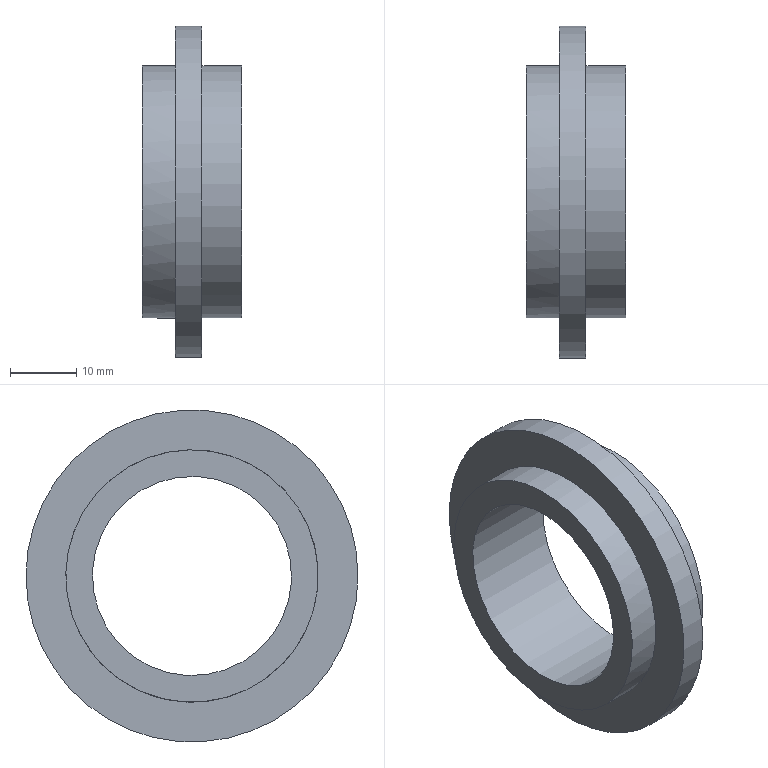Component | NX | XIAODANGYOUHUAN | 1 solid | 8 faces | box 15 x 50 x 50 mm | volume 9726 mm3 | cylinder 4 | plane 4 | commonest cylinder face diameters 38 x2 30 x1 50 x1
STEP:
#1=CARTESIAN_POINT('',(0.,0.,0.));
#2=DIRECTION('',(0.,0.,1.));
#3=DIRECTION('',(1.,0.,0.));
#4=AXIS2_PLACEMENT_3D('',#1,#2,#3);
#5=CARTESIAN_POINT('',(68.,18.801,-90.745));
#6=VERTEX_POINT('',#5);
#7=CARTESIAN_POINT('',(68.,0.,-88.));
#8=DIRECTION('',(1.,0.,0.));
#9=DIRECTION('',(0.,0.9895,-0.1445));
#10=AXIS2_PLACEMENT_3D('',#7,#8,#9);
#11=CIRCLE('',#10,19.);
#12=CARTESIAN_POINT('',(83.,0.,-88.));
#13=DIRECTION('',(-1.,0.,0.));
#14=DIRECTION('',(0.,0.1445,0.9895));
#15=AXIS2_PLACEMENT_3D('',#12,#13,#14);
#16=CYLINDRICAL_SURFACE('',#15,19.);
#17=CARTESIAN_POINT('',(7.854,15.));
#18=DIRECTION('',(-1.,0.));
#19=VECTOR('',#18,1.);
#20=LINE('',#17,#19);
#21=(GEOMETRIC_REPRESENTATION_CONTEXT(2)PARAMETRIC_REPRESENTATION_CONTEXT()REPRESENTATION_CONTEXT('',''));
#22=DEFINITIONAL_REPRESENTATION('',(#20),#21);
#23=PCURVE('',#16,#22);
#24=CARTESIAN_POINT('',(68.,0.,-88.));
#25=DIRECTION('',(1.,0.,0.));
#26=DIRECTION('',(0.,-0.1445,-0.9895));
#27=AXIS2_PLACEMENT_3D('',#24,#25,#26);
#28=PLANE('',#27);
#29=CARTESIAN_POINT('',(0.,0.));
#30=DIRECTION('',(0.,1.));
#31=AXIS2_PLACEMENT_2D('',#29,#30);
#32=CIRCLE('',#31,19.);
#33=(GEOMETRIC_REPRESENTATION_CONTEXT(2)PARAMETRIC_REPRESENTATION_CONTEXT()REPRESENTATION_CONTEXT('',''));
#34=DEFINITIONAL_REPRESENTATION('',(#32),#33);
#35=PCURVE('',#28,#34);
#36=SURFACE_CURVE('',#11,(#23,#35),.PCURVE_S1.);
#37=EDGE_CURVE('',#6,#6,#36,.T.);
#38=ORIENTED_EDGE('',*,*,#37,.T.);
#39=CARTESIAN_POINT('',(73.,18.801,-90.745));
#40=VERTEX_POINT('',#39);
#41=CARTESIAN_POINT('',(73.,18.801,-90.745));
#42=CARTESIAN_POINT('',(68.,18.801,-90.745));
#43=B_SPLINE_CURVE_WITH_KNOTS('',1,(#41,#42),.UNSPECIFIED.,.F.,.F.,(2,2),(10.,15.),.PIECEWISE_BEZIER_KNOTS.);
#44=CARTESIAN_POINT('',(1.571,0.));
#45=DIRECTION('',(0.,1.));
#46=VECTOR('',#45,1.);
#47=LINE('',#44,#46);
#48=(GEOMETRIC_REPRESENTATION_CONTEXT(2)PARAMETRIC_REPRESENTATION_CONTEXT()REPRESENTATION_CONTEXT('',''));
#49=DEFINITIONAL_REPRESENTATION('',(#47),#48);
#50=PCURVE('',#16,#49);
#51=CARTESIAN_POINT('',(7.854,0.));
#52=DIRECTION('',(0.,1.));
#53=VECTOR('',#52,1.);
#54=LINE('',#51,#53);
#55=(GEOMETRIC_REPRESENTATION_CONTEXT(2)PARAMETRIC_REPRESENTATION_CONTEXT()REPRESENTATION_CONTEXT('',''));
#56=DEFINITIONAL_REPRESENTATION('',(#54),#55);
#57=PCURVE('',#16,#56);
#58=SEAM_CURVE('',#43,(#50,#57),.PCURVE_S1.);
#59=EDGE_CURVE('',#40,#6,#58,.T.);
#60=ORIENTED_EDGE('',*,*,#59,.F.);
#61=CARTESIAN_POINT('',(73.,-2.745,-106.801));
#62=VERTEX_POINT('',#61);
#63=CARTESIAN_POINT('',(73.,0.,-88.));
#64=DIRECTION('',(1.,0.,0.));
#65=DIRECTION('',(0.,-0.1445,-0.9895));
#66=AXIS2_PLACEMENT_3D('',#63,#64,#65);
#67=CIRCLE('',#66,19.);
#68=CARTESIAN_POINT('',(3.142,10.));
#69=DIRECTION('',(-1.,0.));
#70=VECTOR('',#69,1.);
#71=LINE('',#68,#70);
#72=(GEOMETRIC_REPRESENTATION_CONTEXT(2)PARAMETRIC_REPRESENTATION_CONTEXT()REPRESENTATION_CONTEXT('',''));
#73=DEFINITIONAL_REPRESENTATION('',(#71),#72);
#74=PCURVE('',#16,#73);
#75=CARTESIAN_POINT('',(73.,0.,-88.));
#76=DIRECTION('',(1.,0.,0.));
#77=DIRECTION('',(0.,-0.1445,-0.9895));
#78=AXIS2_PLACEMENT_3D('',#75,#76,#77);
#79=PLANE('',#78);
#80=CARTESIAN_POINT('',(0.,0.));
#81=DIRECTION('',(1.,0.));
#82=AXIS2_PLACEMENT_2D('',#80,#81);
#83=CIRCLE('',#82,19.);
#84=(GEOMETRIC_REPRESENTATION_CONTEXT(2)PARAMETRIC_REPRESENTATION_CONTEXT()REPRESENTATION_CONTEXT('',''));
#85=DEFINITIONAL_REPRESENTATION('',(#83),#84);
#86=PCURVE('',#79,#85);
#87=SURFACE_CURVE('',#67,(#74,#86),.PCURVE_S1.);
#88=EDGE_CURVE('',#62,#40,#87,.T.);
#89=ORIENTED_EDGE('',*,*,#88,.F.);
#90=CARTESIAN_POINT('',(73.,0.,-88.));
#91=DIRECTION('',(1.,0.,0.));
#92=DIRECTION('',(0.,-0.1445,-0.9895));
#93=AXIS2_PLACEMENT_3D('',#90,#91,#92);
#94=CIRCLE('',#93,19.);
#95=CARTESIAN_POINT('',(9.425,10.));
#96=DIRECTION('',(-1.,0.));
#97=VECTOR('',#96,1.);
#98=LINE('',#95,#97);
#99=(GEOMETRIC_REPRESENTATION_CONTEXT(2)PARAMETRIC_REPRESENTATION_CONTEXT()REPRESENTATION_CONTEXT('',''));
#100=DEFINITIONAL_REPRESENTATION('',(#98),#99);
#101=PCURVE('',#16,#100);
#102=CARTESIAN_POINT('',(0.,0.));
#103=DIRECTION('',(1.,0.));
#104=AXIS2_PLACEMENT_2D('',#102,#103);
#105=CIRCLE('',#104,19.);
#106=(GEOMETRIC_REPRESENTATION_CONTEXT(2)PARAMETRIC_REPRESENTATION_CONTEXT()REPRESENTATION_CONTEXT('',''));
#107=DEFINITIONAL_REPRESENTATION('',(#105),#106);
#108=PCURVE('',#79,#107);
#109=SURFACE_CURVE('',#94,(#101,#108),.PCURVE_S1.);
#110=EDGE_CURVE('',#40,#62,#109,.T.);
#111=ORIENTED_EDGE('',*,*,#110,.F.);
#112=ORIENTED_EDGE('',*,*,#59,.T.);
#113=EDGE_LOOP('',(#38,#60,#89,#111,#112));
#114=FACE_BOUND('',#113,.T.);
#115=ADVANCED_FACE('',(#114),#16,.T.);
#116=CARTESIAN_POINT('',(77.,18.801,-90.745));
#117=VERTEX_POINT('',#116);
#118=CARTESIAN_POINT('',(77.,0.,-88.));
#119=DIRECTION('',(1.,0.,0.));
#120=DIRECTION('',(0.,0.9895,-0.1445));
#121=AXIS2_PLACEMENT_3D('',#118,#119,#120);
#122=CIRCLE('',#121,19.);
#123=CARTESIAN_POINT('',(83.,0.,-88.));
#124=DIRECTION('',(-1.,0.,0.));
#125=DIRECTION('',(0.,0.1445,0.9895));
#126=AXIS2_PLACEMENT_3D('',#123,#124,#125);
#127=CYLINDRICAL_SURFACE('',#126,19.);
#128=CARTESIAN_POINT('',(7.854,6.));
#129=DIRECTION('',(-1.,0.));
#130=VECTOR('',#129,1.);
#131=LINE('',#128,#130);
#132=(GEOMETRIC_REPRESENTATION_CONTEXT(2)PARAMETRIC_REPRESENTATION_CONTEXT()REPRESENTATION_CONTEXT('',''));
#133=DEFINITIONAL_REPRESENTATION('',(#131),#132);
#134=PCURVE('',#127,#133);
#135=CARTESIAN_POINT('',(77.,0.,-88.));
#136=DIRECTION('',(1.,0.,0.));
#137=DIRECTION('',(0.,-0.1445,-0.9895));
#138=AXIS2_PLACEMENT_3D('',#135,#136,#137);
#139=PLANE('',#138);
#140=CARTESIAN_POINT('',(0.,0.));
#141=DIRECTION('',(0.,1.));
#142=AXIS2_PLACEMENT_2D('',#140,#141);
#143=CIRCLE('',#142,19.);
#144=(GEOMETRIC_REPRESENTATION_CONTEXT(2)PARAMETRIC_REPRESENTATION_CONTEXT()REPRESENTATION_CONTEXT('',''));
#145=DEFINITIONAL_REPRESENTATION('',(#143),#144);
#146=PCURVE('',#139,#145);
#147=SURFACE_CURVE('',#122,(#134,#146),.PCURVE_S1.);
#148=EDGE_CURVE('',#117,#117,#147,.T.);
#149=ORIENTED_EDGE('',*,*,#148,.T.);
#150=CARTESIAN_POINT('',(83.,18.801,-90.745));
#151=VERTEX_POINT('',#150);
#152=CARTESIAN_POINT('',(83.,18.801,-90.745));
#153=CARTESIAN_POINT('',(77.,18.801,-90.745));
#154=B_SPLINE_CURVE_WITH_KNOTS('',1,(#152,#153),.UNSPECIFIED.,.F.,.F.,(2,2),(0.,6.),.PIECEWISE_BEZIER_KNOTS.);
#155=CARTESIAN_POINT('',(1.571,0.));
#156=DIRECTION('',(0.,1.));
#157=VECTOR('',#156,1.);
#158=LINE('',#155,#157);
#159=(GEOMETRIC_REPRESENTATION_CONTEXT(2)PARAMETRIC_REPRESENTATION_CONTEXT()REPRESENTATION_CONTEXT('',''));
#160=DEFINITIONAL_REPRESENTATION('',(#158),#159);
#161=PCURVE('',#127,#160);
#162=CARTESIAN_POINT('',(7.854,0.));
#163=DIRECTION('',(0.,1.));
#164=VECTOR('',#163,1.);
#165=LINE('',#162,#164);
#166=(GEOMETRIC_REPRESENTATION_CONTEXT(2)PARAMETRIC_REPRESENTATION_CONTEXT()REPRESENTATION_CONTEXT('',''));
#167=DEFINITIONAL_REPRESENTATION('',(#165),#166);
#168=PCURVE('',#127,#167);
#169=SEAM_CURVE('',#154,(#161,#168),.PCURVE_S1.);
#170=EDGE_CURVE('',#151,#117,#169,.T.);
#171=ORIENTED_EDGE('',*,*,#170,.F.);
#172=CARTESIAN_POINT('',(83.,0.,-88.));
#173=DIRECTION('',(1.,0.,0.));
#174=DIRECTION('',(0.,0.9895,-0.1445));
#175=AXIS2_PLACEMENT_3D('',#172,#173,#174);
#176=CIRCLE('',#175,19.);
#177=CARTESIAN_POINT('',(7.854,0.));
#178=DIRECTION('',(-1.,0.));
#179=VECTOR('',#178,1.);
#180=LINE('',#177,#179);
#181=(GEOMETRIC_REPRESENTATION_CONTEXT(2)PARAMETRIC_REPRESENTATION_CONTEXT()REPRESENTATION_CONTEXT('',''));
#182=DEFINITIONAL_REPRESENTATION('',(#180),#181);
#183=PCURVE('',#127,#182);
#184=CARTESIAN_POINT('',(83.,0.,-88.));
#185=DIRECTION('',(1.,0.,0.));
#186=DIRECTION('',(0.,-0.1445,-0.9895));
#187=AXIS2_PLACEMENT_3D('',#184,#185,#186);
#188=PLANE('',#187);
#189=CARTESIAN_POINT('',(0.,0.));
#190=DIRECTION('',(0.,1.));
#191=AXIS2_PLACEMENT_2D('',#189,#190);
#192=CIRCLE('',#191,19.);
#193=(GEOMETRIC_REPRESENTATION_CONTEXT(2)PARAMETRIC_REPRESENTATION_CONTEXT()REPRESENTATION_CONTEXT('',''));
#194=DEFINITIONAL_REPRESENTATION('',(#192),#193);
#195=PCURVE('',#188,#194);
#196=SURFACE_CURVE('',#176,(#183,#195),.PCURVE_S1.);
#197=EDGE_CURVE('',#151,#151,#196,.T.);
#198=ORIENTED_EDGE('',*,*,#197,.F.);
#199=ORIENTED_EDGE('',*,*,#170,.T.);
#200=EDGE_LOOP('',(#149,#171,#198,#199));
#201=FACE_BOUND('',#200,.T.);
#202=ADVANCED_FACE('',(#201),#127,.T.);
#203=CARTESIAN_POINT('',(83.,14.843,-90.167));
#204=VERTEX_POINT('',#203);
#205=CARTESIAN_POINT('',(83.,0.,-88.));
#206=DIRECTION('',(1.,0.,0.));
#207=DIRECTION('',(0.,0.9895,-0.1445));
#208=AXIS2_PLACEMENT_3D('',#205,#206,#207);
#209=CIRCLE('',#208,15.);
#210=CARTESIAN_POINT('',(83.,0.,-88.));
#211=DIRECTION('',(-1.,0.,0.));
#212=DIRECTION('',(0.,0.1445,0.9895));
#213=AXIS2_PLACEMENT_3D('',#210,#211,#212);
#214=CYLINDRICAL_SURFACE('',#213,15.);
#215=CARTESIAN_POINT('',(7.854,0.));
#216=DIRECTION('',(-1.,0.));
#217=VECTOR('',#216,1.);
#218=LINE('',#215,#217);
#219=(GEOMETRIC_REPRESENTATION_CONTEXT(2)PARAMETRIC_REPRESENTATION_CONTEXT()REPRESENTATION_CONTEXT('',''));
#220=DEFINITIONAL_REPRESENTATION('',(#218),#219);
#221=PCURVE('',#214,#220);
#222=CARTESIAN_POINT('',(0.,0.));
#223=DIRECTION('',(0.,1.));
#224=AXIS2_PLACEMENT_2D('',#222,#223);
#225=CIRCLE('',#224,15.);
#226=(GEOMETRIC_REPRESENTATION_CONTEXT(2)PARAMETRIC_REPRESENTATION_CONTEXT()REPRESENTATION_CONTEXT('',''));
#227=DEFINITIONAL_REPRESENTATION('',(#225),#226);
#228=PCURVE('',#188,#227);
#229=SURFACE_CURVE('',#209,(#221,#228),.PCURVE_S1.);
#230=EDGE_CURVE('',#204,#204,#229,.T.);
#231=ORIENTED_EDGE('',*,*,#230,.F.);
#232=CARTESIAN_POINT('',(68.,14.843,-90.167));
#233=VERTEX_POINT('',#232);
#234=CARTESIAN_POINT('',(83.,14.843,-90.167));
#235=CARTESIAN_POINT('',(68.,14.843,-90.167));
#236=B_SPLINE_CURVE_WITH_KNOTS('',1,(#234,#235),.UNSPECIFIED.,.F.,.F.,(2,2),(0.,15.),.PIECEWISE_BEZIER_KNOTS.);
#237=CARTESIAN_POINT('',(7.854,0.));
#238=DIRECTION('',(0.,1.));
#239=VECTOR('',#238,1.);
#240=LINE('',#237,#239);
#241=(GEOMETRIC_REPRESENTATION_CONTEXT(2)PARAMETRIC_REPRESENTATION_CONTEXT()REPRESENTATION_CONTEXT('',''));
#242=DEFINITIONAL_REPRESENTATION('',(#240),#241);
#243=PCURVE('',#214,#242);
#244=CARTESIAN_POINT('',(1.571,0.));
#245=DIRECTION('',(0.,1.));
#246=VECTOR('',#245,1.);
#247=LINE('',#244,#246);
#248=(GEOMETRIC_REPRESENTATION_CONTEXT(2)PARAMETRIC_REPRESENTATION_CONTEXT()REPRESENTATION_CONTEXT('',''));
#249=DEFINITIONAL_REPRESENTATION('',(#247),#248);
#250=PCURVE('',#214,#249);
#251=SEAM_CURVE('',#236,(#243,#250),.PCURVE_S1.);
#252=EDGE_CURVE('',#204,#233,#251,.T.);
#253=ORIENTED_EDGE('',*,*,#252,.T.);
#254=CARTESIAN_POINT('',(68.,0.,-88.));
#255=DIRECTION('',(1.,0.,0.));
#256=DIRECTION('',(0.,0.9895,-0.1445));
#257=AXIS2_PLACEMENT_3D('',#254,#255,#256);
#258=CIRCLE('',#257,15.);
#259=CARTESIAN_POINT('',(7.854,15.));
#260=DIRECTION('',(-1.,0.));
#261=VECTOR('',#260,1.);
#262=LINE('',#259,#261);
#263=(GEOMETRIC_REPRESENTATION_CONTEXT(2)PARAMETRIC_REPRESENTATION_CONTEXT()REPRESENTATION_CONTEXT('',''));
#264=DEFINITIONAL_REPRESENTATION('',(#262),#263);
#265=PCURVE('',#214,#264);
#266=CARTESIAN_POINT('',(0.,0.));
#267=DIRECTION('',(0.,1.));
#268=AXIS2_PLACEMENT_2D('',#266,#267);
#269=CIRCLE('',#268,15.);
#270=(GEOMETRIC_REPRESENTATION_CONTEXT(2)PARAMETRIC_REPRESENTATION_CONTEXT()REPRESENTATION_CONTEXT('',''));
#271=DEFINITIONAL_REPRESENTATION('',(#269),#270);
#272=PCURVE('',#28,#271);
#273=SURFACE_CURVE('',#258,(#265,#272),.PCURVE_S1.);
#274=EDGE_CURVE('',#233,#233,#273,.T.);
#275=ORIENTED_EDGE('',*,*,#274,.T.);
#276=ORIENTED_EDGE('',*,*,#252,.F.);
#277=EDGE_LOOP('',(#231,#253,#275,#276));
#278=FACE_BOUND('',#277,.F.);
#279=ADVANCED_FACE('',(#278),#214,.F.);
#280=ORIENTED_EDGE('',*,*,#197,.T.);
#281=EDGE_LOOP('',(#280));
#282=FACE_BOUND('',#281,.T.);
#283=ORIENTED_EDGE('',*,*,#230,.F.);
#284=EDGE_LOOP('',(#283));
#285=FACE_BOUND('',#284,.T.);
#286=ADVANCED_FACE('',(#282,#285),#188,.T.);
#287=ORIENTED_EDGE('',*,*,#37,.F.);
#288=EDGE_LOOP('',(#287));
#289=FACE_BOUND('',#288,.T.);
#290=ORIENTED_EDGE('',*,*,#274,.T.);
#291=EDGE_LOOP('',(#290));
#292=FACE_BOUND('',#291,.T.);
#293=ADVANCED_FACE('',(#289,#292),#28,.F.);
#294=CARTESIAN_POINT('',(77.,24.738,-91.612));
#295=VERTEX_POINT('',#294);
#296=CARTESIAN_POINT('',(77.,0.,-88.));
#297=DIRECTION('',(1.,0.,0.));
#298=DIRECTION('',(0.,0.9895,-0.1445));
#299=AXIS2_PLACEMENT_3D('',#296,#297,#298);
#300=CIRCLE('',#299,25.);
#301=CARTESIAN_POINT('',(77.,0.,-88.));
#302=DIRECTION('',(-1.,0.,0.));
#303=DIRECTION('',(0.,0.1445,0.9895));
#304=AXIS2_PLACEMENT_3D('',#301,#302,#303);
#305=CYLINDRICAL_SURFACE('',#304,25.);
#306=CARTESIAN_POINT('',(7.854,0.));
#307=DIRECTION('',(-1.,0.));
#308=VECTOR('',#307,1.);
#309=LINE('',#306,#308);
#310=(GEOMETRIC_REPRESENTATION_CONTEXT(2)PARAMETRIC_REPRESENTATION_CONTEXT()REPRESENTATION_CONTEXT('',''));
#311=DEFINITIONAL_REPRESENTATION('',(#309),#310);
#312=PCURVE('',#305,#311);
#313=CARTESIAN_POINT('',(0.,0.));
#314=DIRECTION('',(0.,1.));
#315=AXIS2_PLACEMENT_2D('',#313,#314);
#316=CIRCLE('',#315,25.);
#317=(GEOMETRIC_REPRESENTATION_CONTEXT(2)PARAMETRIC_REPRESENTATION_CONTEXT()REPRESENTATION_CONTEXT('',''));
#318=DEFINITIONAL_REPRESENTATION('',(#316),#317);
#319=PCURVE('',#139,#318);
#320=SURFACE_CURVE('',#300,(#312,#319),.PCURVE_S1.);
#321=EDGE_CURVE('',#295,#295,#320,.T.);
#322=ORIENTED_EDGE('',*,*,#321,.F.);
#323=CARTESIAN_POINT('',(73.,24.738,-91.612));
#324=VERTEX_POINT('',#323);
#325=CARTESIAN_POINT('',(77.,24.738,-91.612));
#326=CARTESIAN_POINT('',(73.,24.738,-91.612));
#327=B_SPLINE_CURVE_WITH_KNOTS('',1,(#325,#326),.UNSPECIFIED.,.F.,.F.,(2,2),(0.,4.),.PIECEWISE_BEZIER_KNOTS.);
#328=CARTESIAN_POINT('',(7.854,0.));
#329=DIRECTION('',(0.,1.));
#330=VECTOR('',#329,1.);
#331=LINE('',#328,#330);
#332=(GEOMETRIC_REPRESENTATION_CONTEXT(2)PARAMETRIC_REPRESENTATION_CONTEXT()REPRESENTATION_CONTEXT('',''));
#333=DEFINITIONAL_REPRESENTATION('',(#331),#332);
#334=PCURVE('',#305,#333);
#335=CARTESIAN_POINT('',(1.571,0.));
#336=DIRECTION('',(0.,1.));
#337=VECTOR('',#336,1.);
#338=LINE('',#335,#337);
#339=(GEOMETRIC_REPRESENTATION_CONTEXT(2)PARAMETRIC_REPRESENTATION_CONTEXT()REPRESENTATION_CONTEXT('',''));
#340=DEFINITIONAL_REPRESENTATION('',(#338),#339);
#341=PCURVE('',#305,#340);
#342=SEAM_CURVE('',#327,(#334,#341),.PCURVE_S1.);
#343=EDGE_CURVE('',#295,#324,#342,.T.);
#344=ORIENTED_EDGE('',*,*,#343,.T.);
#345=CARTESIAN_POINT('',(73.,0.,-88.));
#346=DIRECTION('',(1.,0.,0.));
#347=DIRECTION('',(0.,0.9895,-0.1445));
#348=AXIS2_PLACEMENT_3D('',#345,#346,#347);
#349=CIRCLE('',#348,25.);
#350=CARTESIAN_POINT('',(7.854,4.));
#351=DIRECTION('',(-1.,0.));
#352=VECTOR('',#351,1.);
#353=LINE('',#350,#352);
#354=(GEOMETRIC_REPRESENTATION_CONTEXT(2)PARAMETRIC_REPRESENTATION_CONTEXT()REPRESENTATION_CONTEXT('',''));
#355=DEFINITIONAL_REPRESENTATION('',(#353),#354);
#356=PCURVE('',#305,#355);
#357=CARTESIAN_POINT('',(0.,0.));
#358=DIRECTION('',(0.,1.));
#359=AXIS2_PLACEMENT_2D('',#357,#358);
#360=CIRCLE('',#359,25.);
#361=(GEOMETRIC_REPRESENTATION_CONTEXT(2)PARAMETRIC_REPRESENTATION_CONTEXT()REPRESENTATION_CONTEXT('',''));
#362=DEFINITIONAL_REPRESENTATION('',(#360),#361);
#363=PCURVE('',#79,#362);
#364=SURFACE_CURVE('',#349,(#356,#363),.PCURVE_S1.);
#365=EDGE_CURVE('',#324,#324,#364,.T.);
#366=ORIENTED_EDGE('',*,*,#365,.T.);
#367=ORIENTED_EDGE('',*,*,#343,.F.);
#368=EDGE_LOOP('',(#322,#344,#366,#367));
#369=FACE_BOUND('',#368,.T.);
#370=ADVANCED_FACE('',(#369),#305,.T.);
#371=ORIENTED_EDGE('',*,*,#321,.T.);
#372=EDGE_LOOP('',(#371));
#373=FACE_BOUND('',#372,.T.);
#374=ORIENTED_EDGE('',*,*,#148,.F.);
#375=EDGE_LOOP('',(#374));
#376=FACE_BOUND('',#375,.T.);
#377=ADVANCED_FACE('',(#373,#376),#139,.T.);
#378=ORIENTED_EDGE('',*,*,#365,.F.);
#379=EDGE_LOOP('',(#378));
#380=FACE_BOUND('',#379,.T.);
#381=ORIENTED_EDGE('',*,*,#88,.T.);
#382=ORIENTED_EDGE('',*,*,#110,.T.);
#383=EDGE_LOOP('',(#381,#382));
#384=FACE_BOUND('',#383,.T.);
#385=ADVANCED_FACE('',(#380,#384),#79,.F.);
#386=CLOSED_SHELL('',(#115,#202,#279,#286,#293,#370,#377,#385));
#387=MANIFOLD_SOLID_BREP('',#386);
#388=(LENGTH_UNIT()NAMED_UNIT(*)SI_UNIT(.MILLI.,.METRE.));
#389=UNCERTAINTY_MEASURE_WITH_UNIT(LENGTH_MEASURE(0.000005),#388,'','');
#390=(NAMED_UNIT(*)PLANE_ANGLE_UNIT()SI_UNIT($,.RADIAN.));
#391=(NAMED_UNIT(*)SI_UNIT($,.STERADIAN.)SOLID_ANGLE_UNIT());
#392=(GEOMETRIC_REPRESENTATION_CONTEXT(3)GLOBAL_UNCERTAINTY_ASSIGNED_CONTEXT((#389))GLOBAL_UNIT_ASSIGNED_CONTEXT((#388,#390,#391))REPRESENTATION_CONTEXT('',''));
#393=ADVANCED_BREP_SHAPE_REPRESENTATION('',(#4,#387),#392);